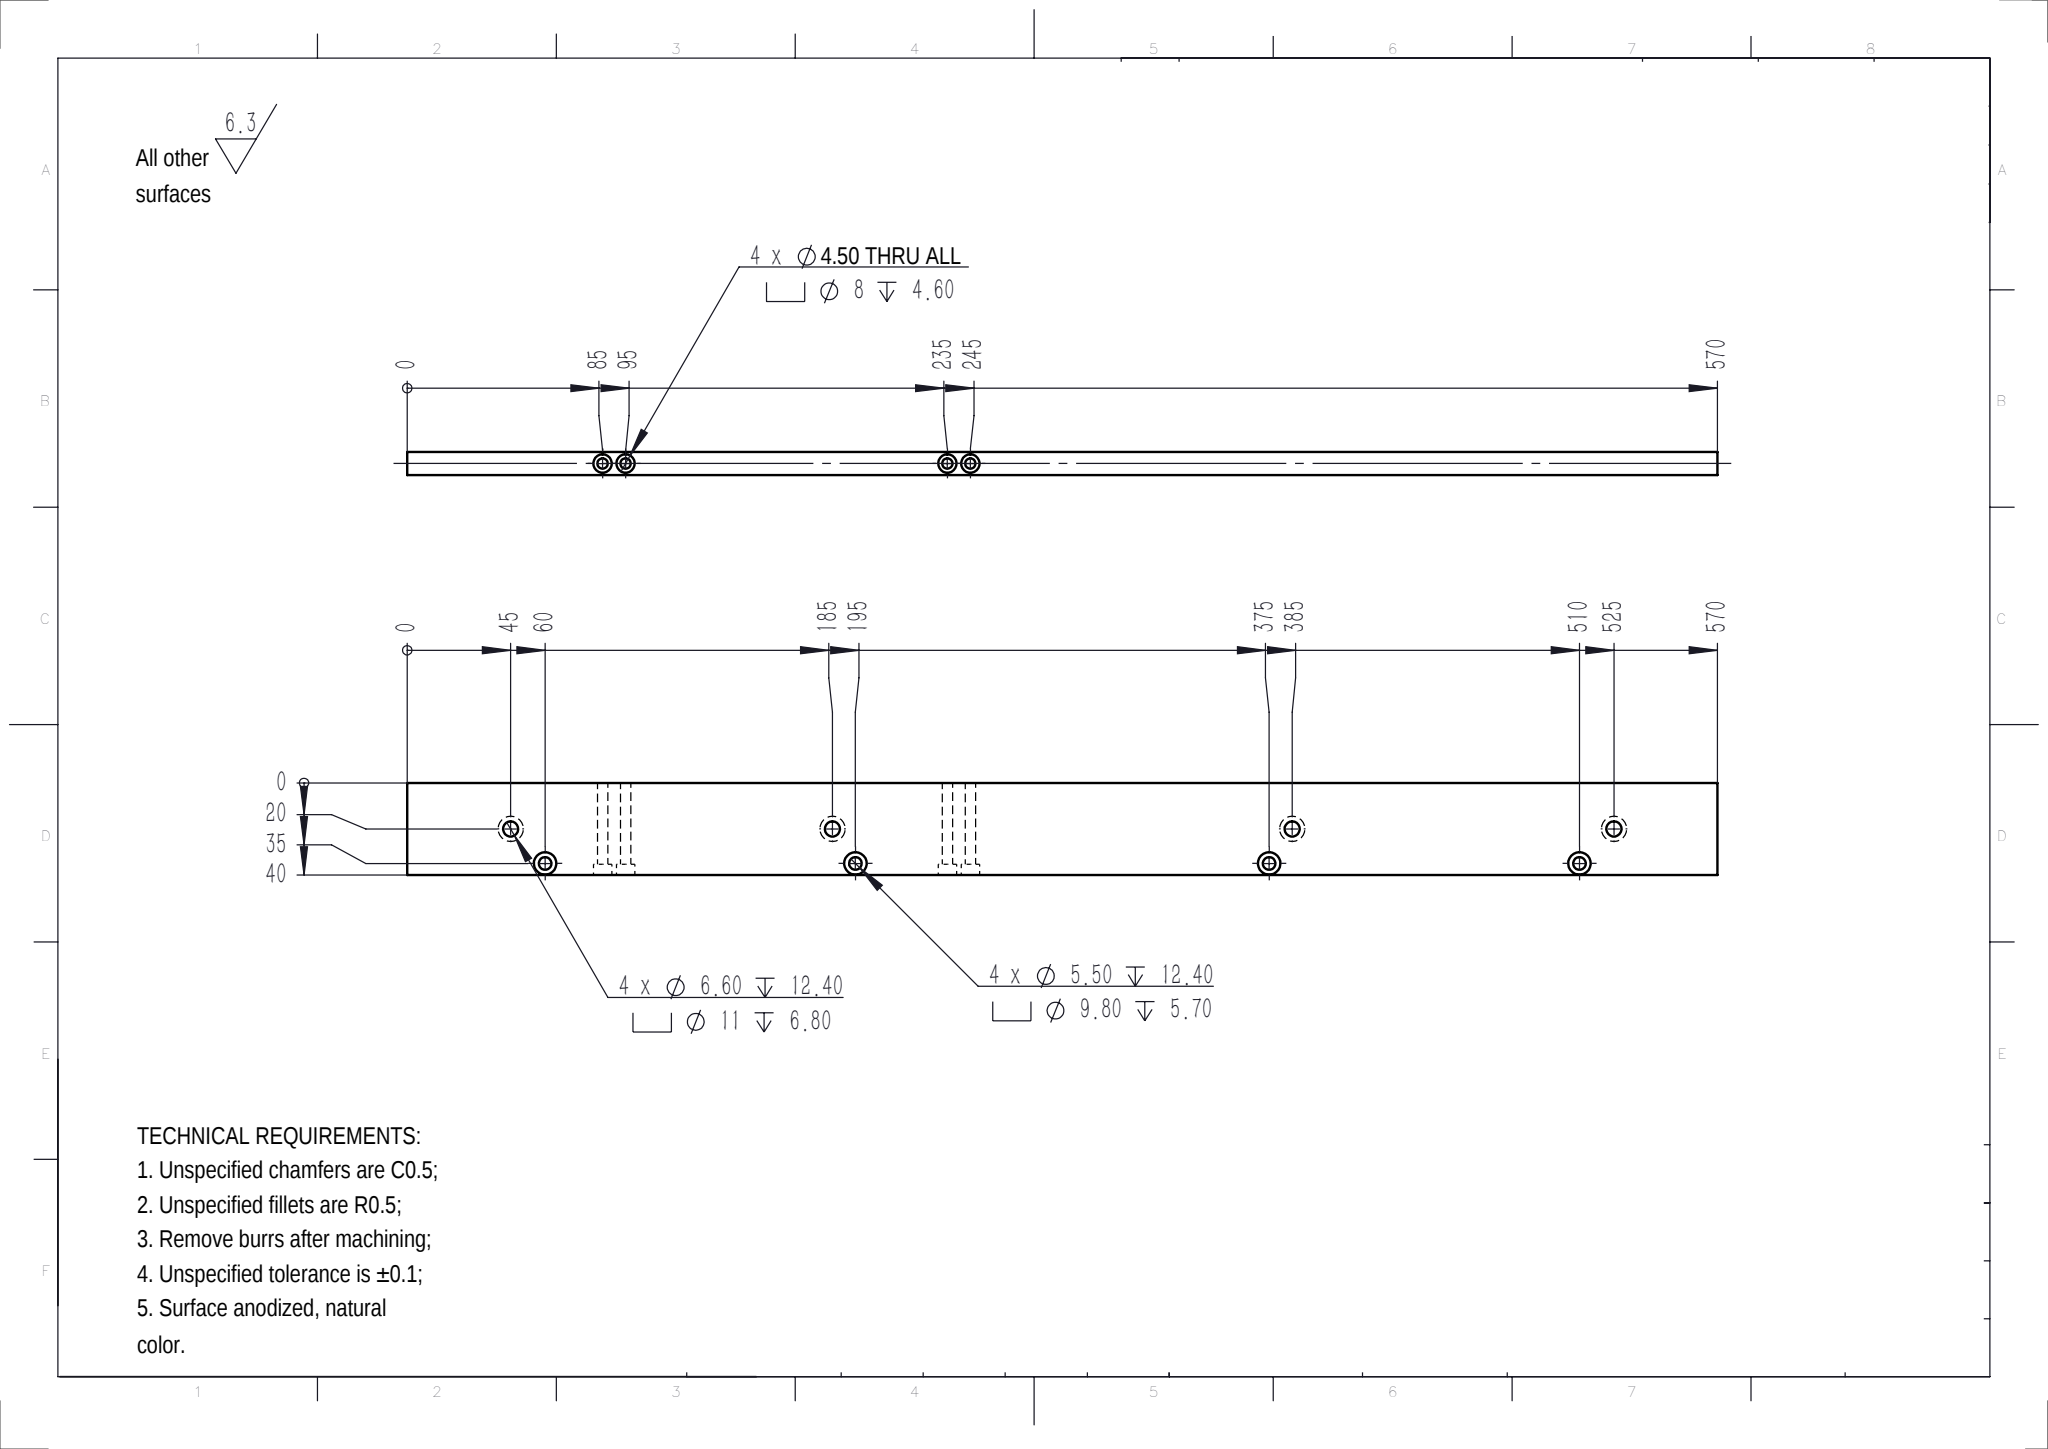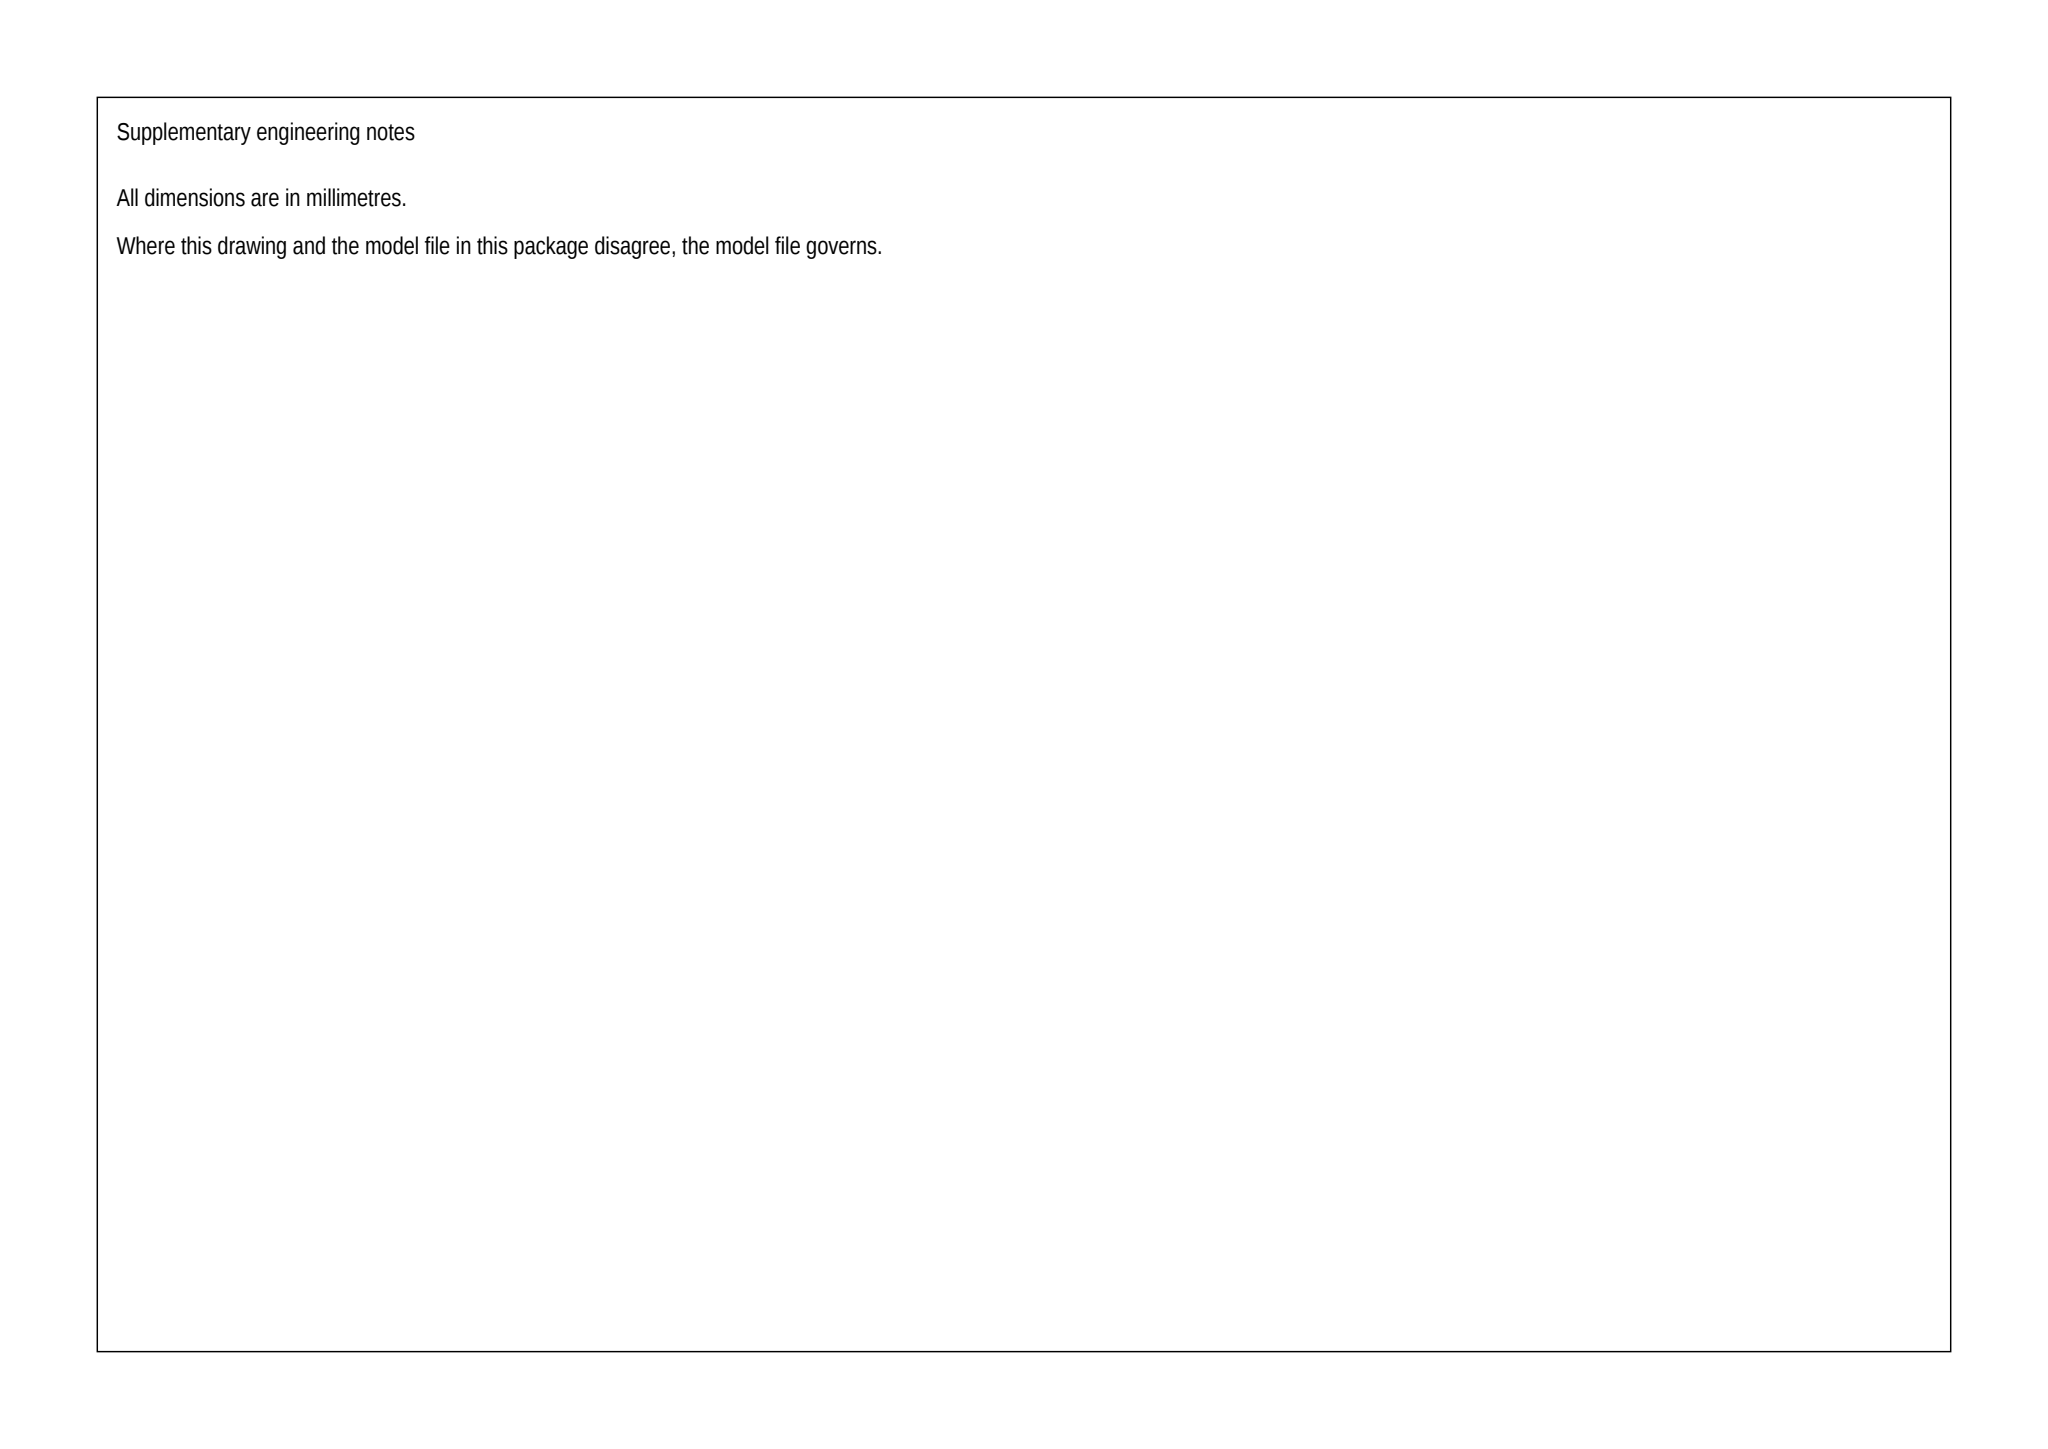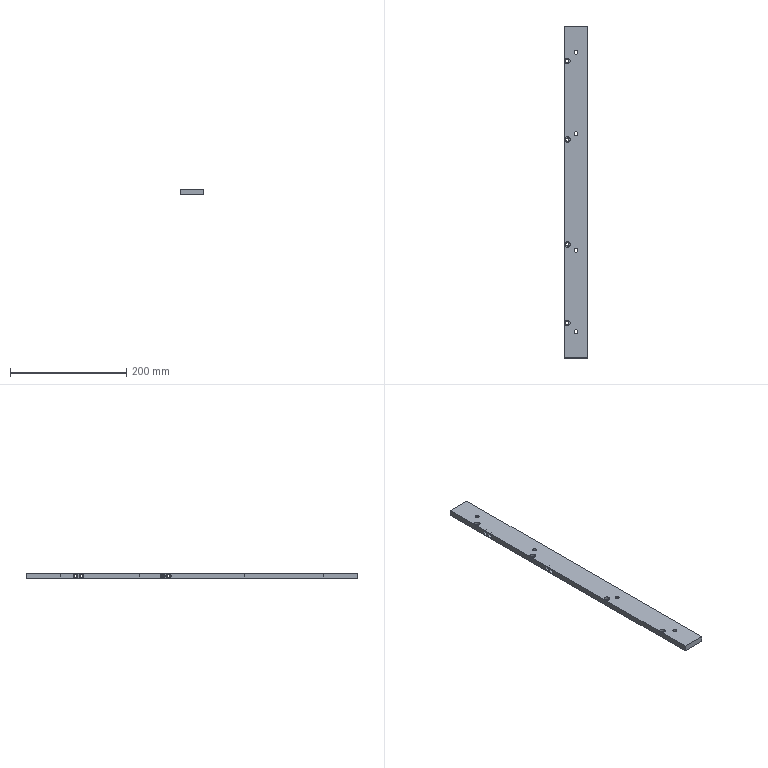Part | SolidWorks | mm | 1 solid | 66 faces | box 40 x 570 x 10 mm | volume 219672 mm3 | cylinder 48 | plane 18 | commonest cylinder face diameters 11 x8 6.6 x8 9.8 x8 5.5 x8 8 x8 4.5 x8
build123d program:
from build123d import *

# Parameters (mm, degrees)
SKETCH1_W                                         = 40
SKETCH1_H                                         = 570
BOSS_EXTRUDE1_DEPTH                               = 10
HOLE_SIZE_ACCORDING_TO_HEXAGON_SOCKET_D           = 4.5
HOLE_SIZE_ACCORDING_TO_HEXAGON_SOCKET_CBORE_D     = 8
HOLE_SIZE_ACCORDING_TO_HEXAGON_SOCKET_CBORE_DEPTH = 4.6
HOLE_SIZE_ACCORDING_TO_HEXAGON_SO_2_D             = 5.5
HOLE_SIZE_ACCORDING_TO_HEXAGON_SO_2_DEPTH         = 12.4
HOLE_SIZE_ACCORDING_TO_HEXAGON_SO_2_CBORE_D       = 9.8
HOLE_SIZE_ACCORDING_TO_HEXAGON_SO_2_CBORE_DEPTH   = 5.7
HOLE_SIZE_ACCORDING_TO_HEXAGON_SO_2_TIP           = 1.652
HOLE_SIZE_ACCORDING_TO_HEXAGON_SO_3_D             = 6.6
HOLE_SIZE_ACCORDING_TO_HEXAGON_SO_3_DEPTH         = 12.4
HOLE_SIZE_ACCORDING_TO_HEXAGON_SO_3_CBORE_D       = 11
HOLE_SIZE_ACCORDING_TO_HEXAGON_SO_3_CBORE_DEPTH   = 6.8
HOLE_SIZE_ACCORDING_TO_HEXAGON_SO_3_TIP           = 1.983


with BuildPart() as part:
    # Sketch1 → Boss-Extrude1 (new body)
    with BuildSketch(Plane.XY):
        Rectangle(SKETCH1_W, SKETCH1_H)
    extrude(amount=BOSS_EXTRUDE1_DEPTH)

    # Hole Size _ according to_ Hexagon Socket (through all)
    with Locations(Plane(origin=(-20, 0, 0), x_dir=(0, 0, -1), z_dir=(-1, 0, 0))):
        with Locations((-5, -50), (-5, -200), (-5, -190), (-5, -40)):
            CounterBoreHole(HOLE_SIZE_ACCORDING_TO_HEXAGON_SOCKET_D / 2, HOLE_SIZE_ACCORDING_TO_HEXAGON_SOCKET_CBORE_D / 2, HOLE_SIZE_ACCORDING_TO_HEXAGON_SOCKET_CBORE_DEPTH)

    # Hole Size _ according to_ Hexagon So 2
    with Locations(Plane.XY.offset(10)):
        with Locations((-15, 225), (-15, 90), (-15, -90), (-15, -225)):
            CounterBoreHole(HOLE_SIZE_ACCORDING_TO_HEXAGON_SO_2_D / 2, HOLE_SIZE_ACCORDING_TO_HEXAGON_SO_2_CBORE_D / 2, HOLE_SIZE_ACCORDING_TO_HEXAGON_SO_2_CBORE_DEPTH, depth=HOLE_SIZE_ACCORDING_TO_HEXAGON_SO_2_DEPTH)
            with Locations((0, 0, -(HOLE_SIZE_ACCORDING_TO_HEXAGON_SO_2_DEPTH + HOLE_SIZE_ACCORDING_TO_HEXAGON_SO_2_TIP / 2))):  # 118° drill point
                Cone(0, HOLE_SIZE_ACCORDING_TO_HEXAGON_SO_2_D / 2, HOLE_SIZE_ACCORDING_TO_HEXAGON_SO_2_TIP, mode=Mode.SUBTRACT)

    # Hole Size _ according to_ Hexagon So 3
    with Locations(Plane(origin=(0, 0, 0), x_dir=(-1, 0, 0), z_dir=(0, 0, -1))):
        with Locations((0, 240), (0, 100), (0, -100), (0, -240)):
            CounterBoreHole(HOLE_SIZE_ACCORDING_TO_HEXAGON_SO_3_D / 2, HOLE_SIZE_ACCORDING_TO_HEXAGON_SO_3_CBORE_D / 2, HOLE_SIZE_ACCORDING_TO_HEXAGON_SO_3_CBORE_DEPTH, depth=HOLE_SIZE_ACCORDING_TO_HEXAGON_SO_3_DEPTH)
            with Locations((0, 0, -(HOLE_SIZE_ACCORDING_TO_HEXAGON_SO_3_DEPTH + HOLE_SIZE_ACCORDING_TO_HEXAGON_SO_3_TIP / 2))):  # 118° drill point
                Cone(0, HOLE_SIZE_ACCORDING_TO_HEXAGON_SO_3_D / 2, HOLE_SIZE_ACCORDING_TO_HEXAGON_SO_3_TIP, mode=Mode.SUBTRACT)


solid = part.part